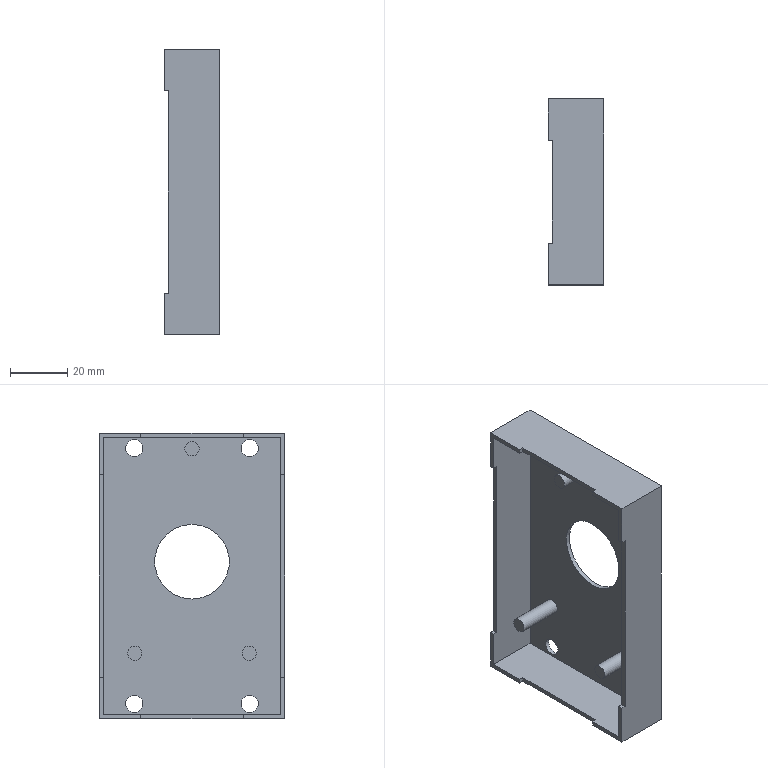Component | NX | HOUSING | 1 solid | 37 faces | volume 18016 mm3 | plane 29 | cylinder 8 | commonest cylinder face diameters 6 x4 5 x3 26.1 x1